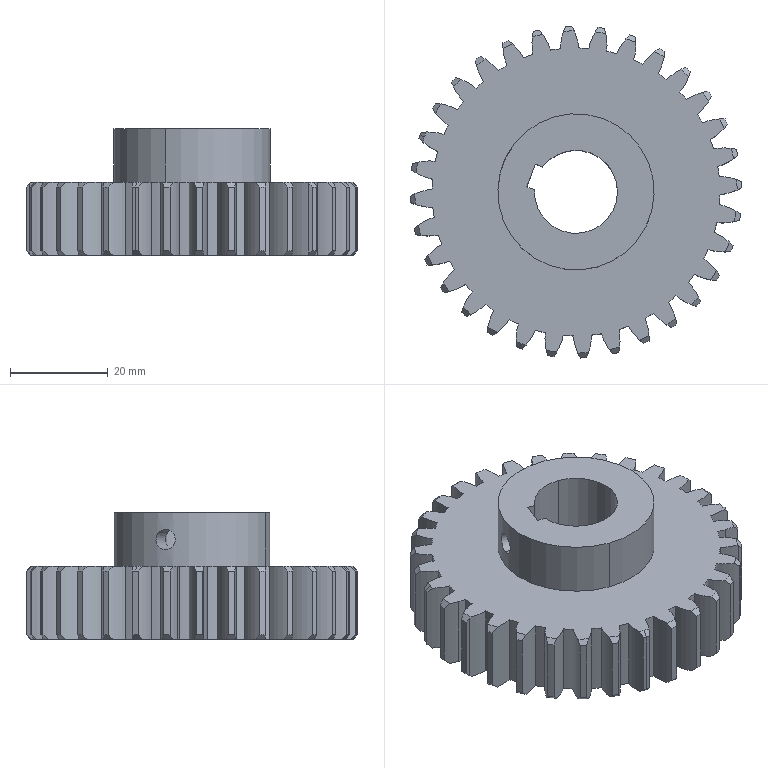Component | SolidWorks | Gear2-1 | 1 solid | 216 faces | volume 49778 mm3 | cylinder 140 | cone 69 | plane 7 | commonest cylinder face diameters 24.155 x68 68 x33 59 x32 17 x3 32 x2 4.2 x2